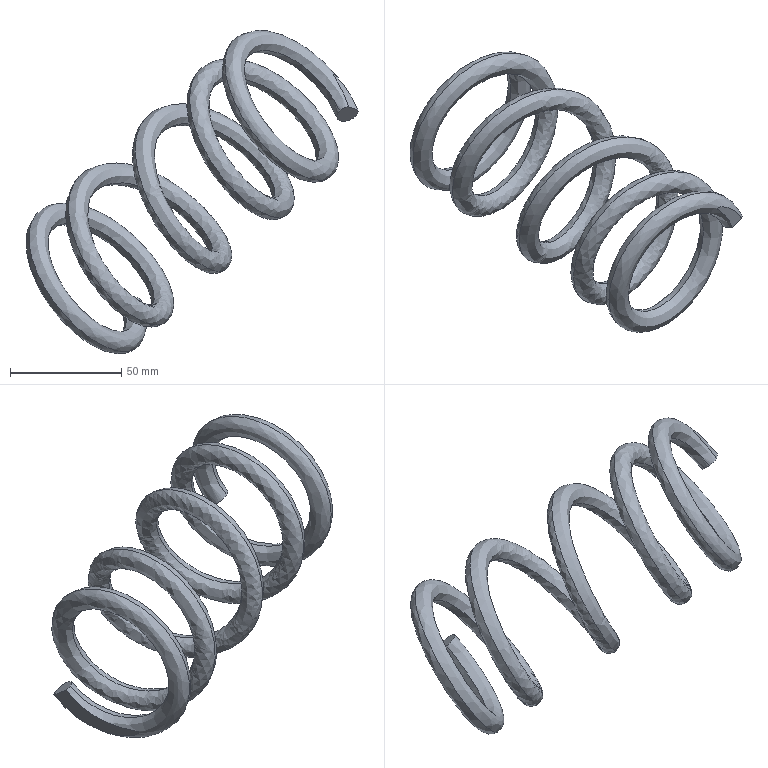Component | SolidWorks | DampingSpring-2 | 1 solid | 6 faces | volume 80277 mm3 | plane 4 | spline 2 | material Chrome Stainless Steel